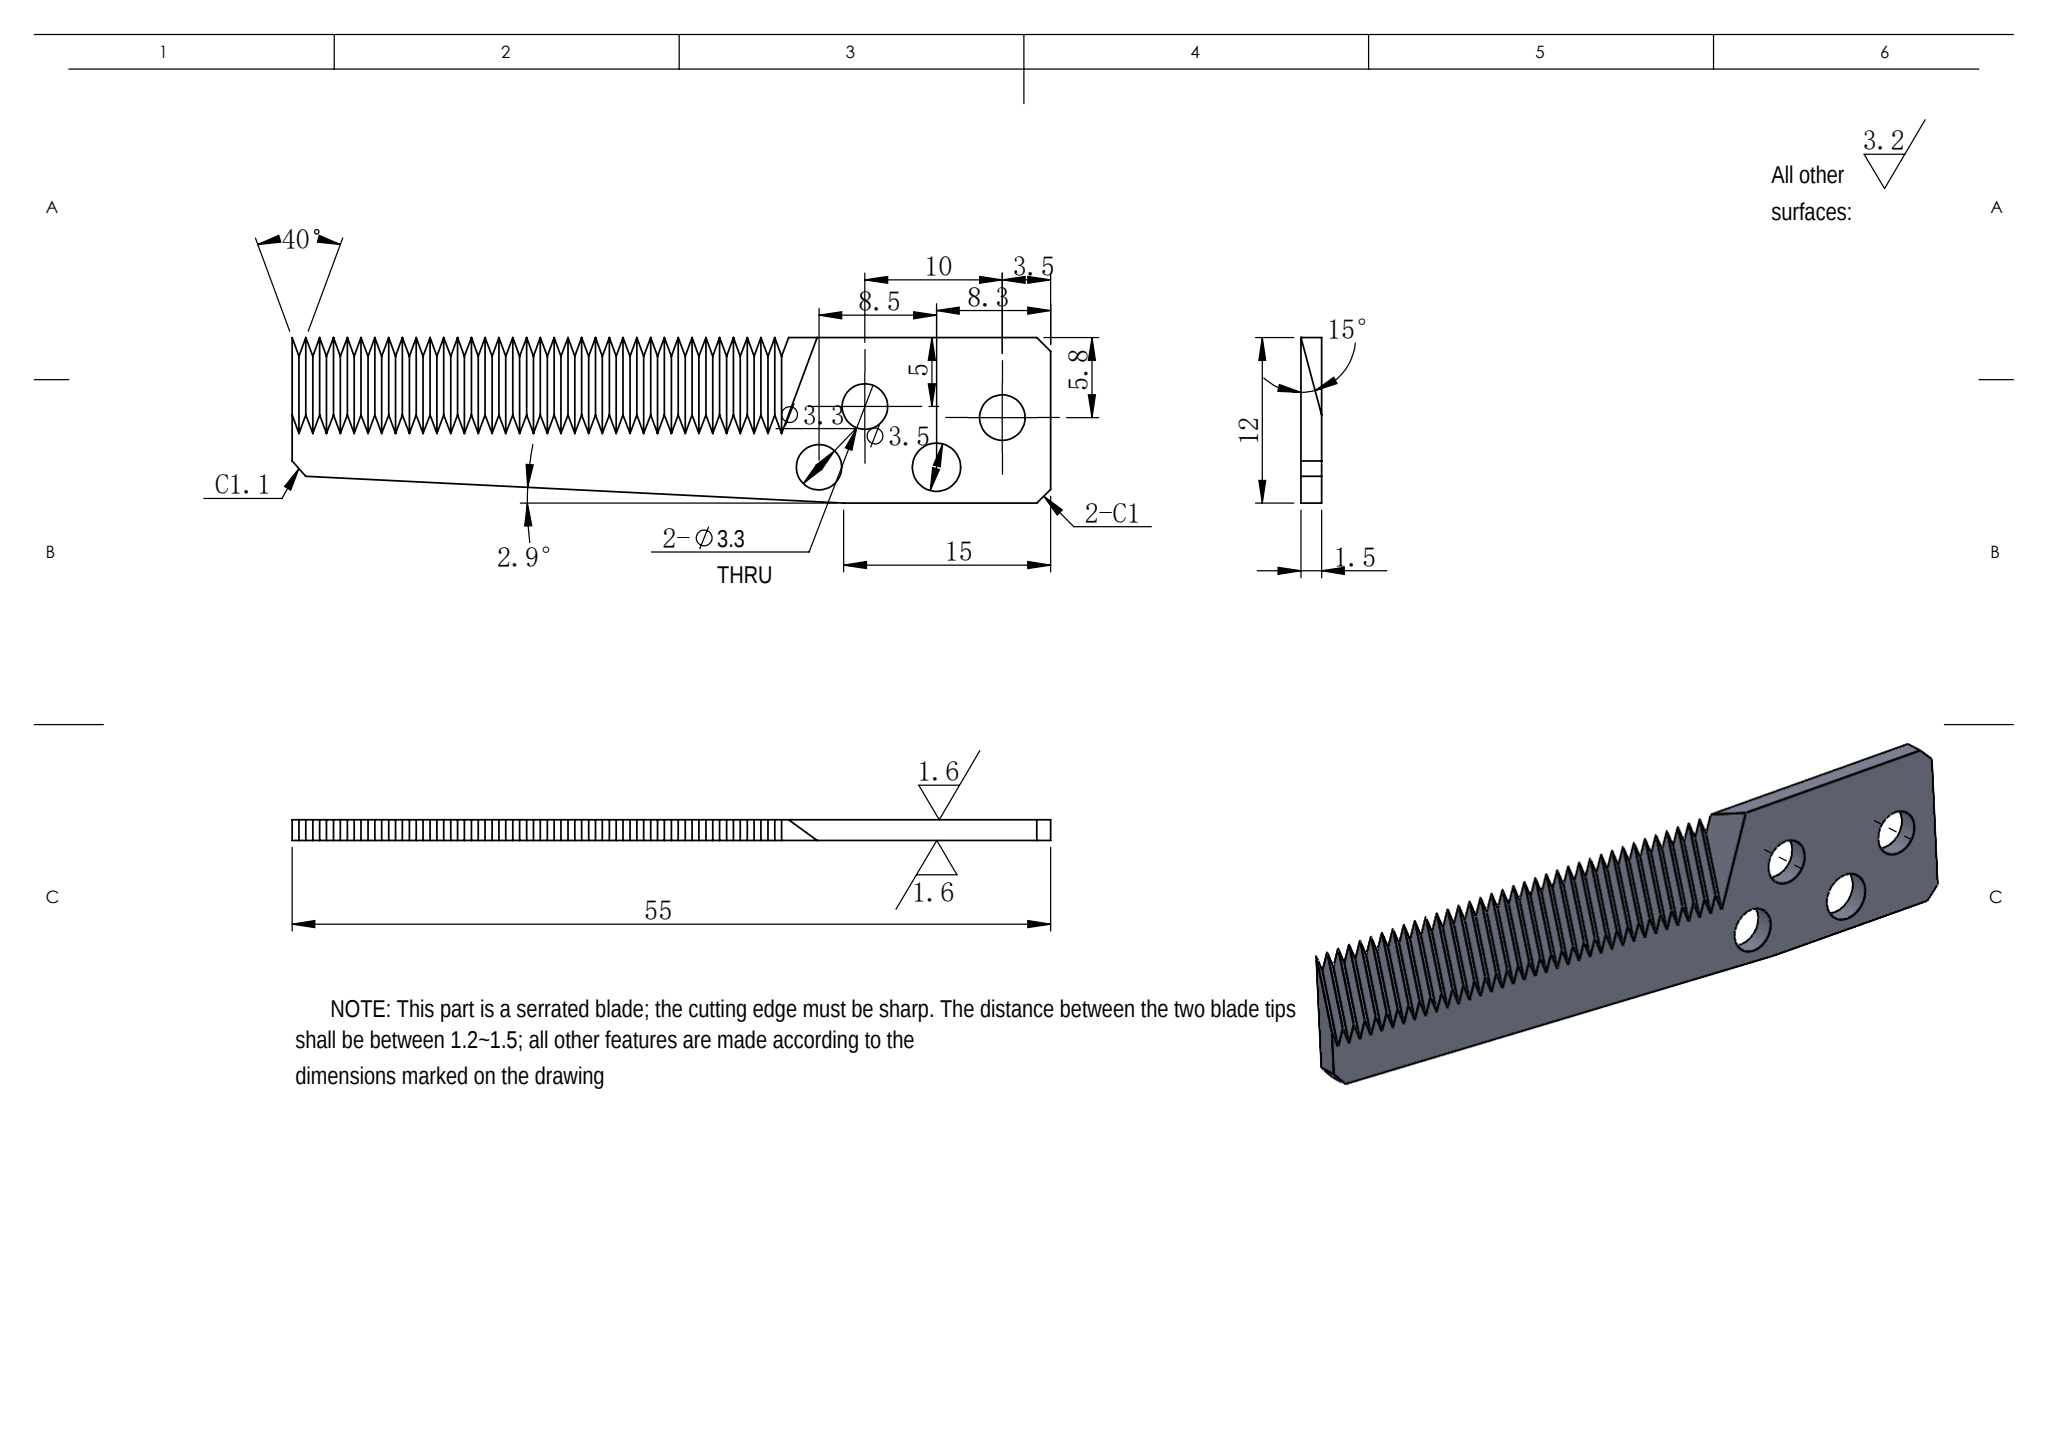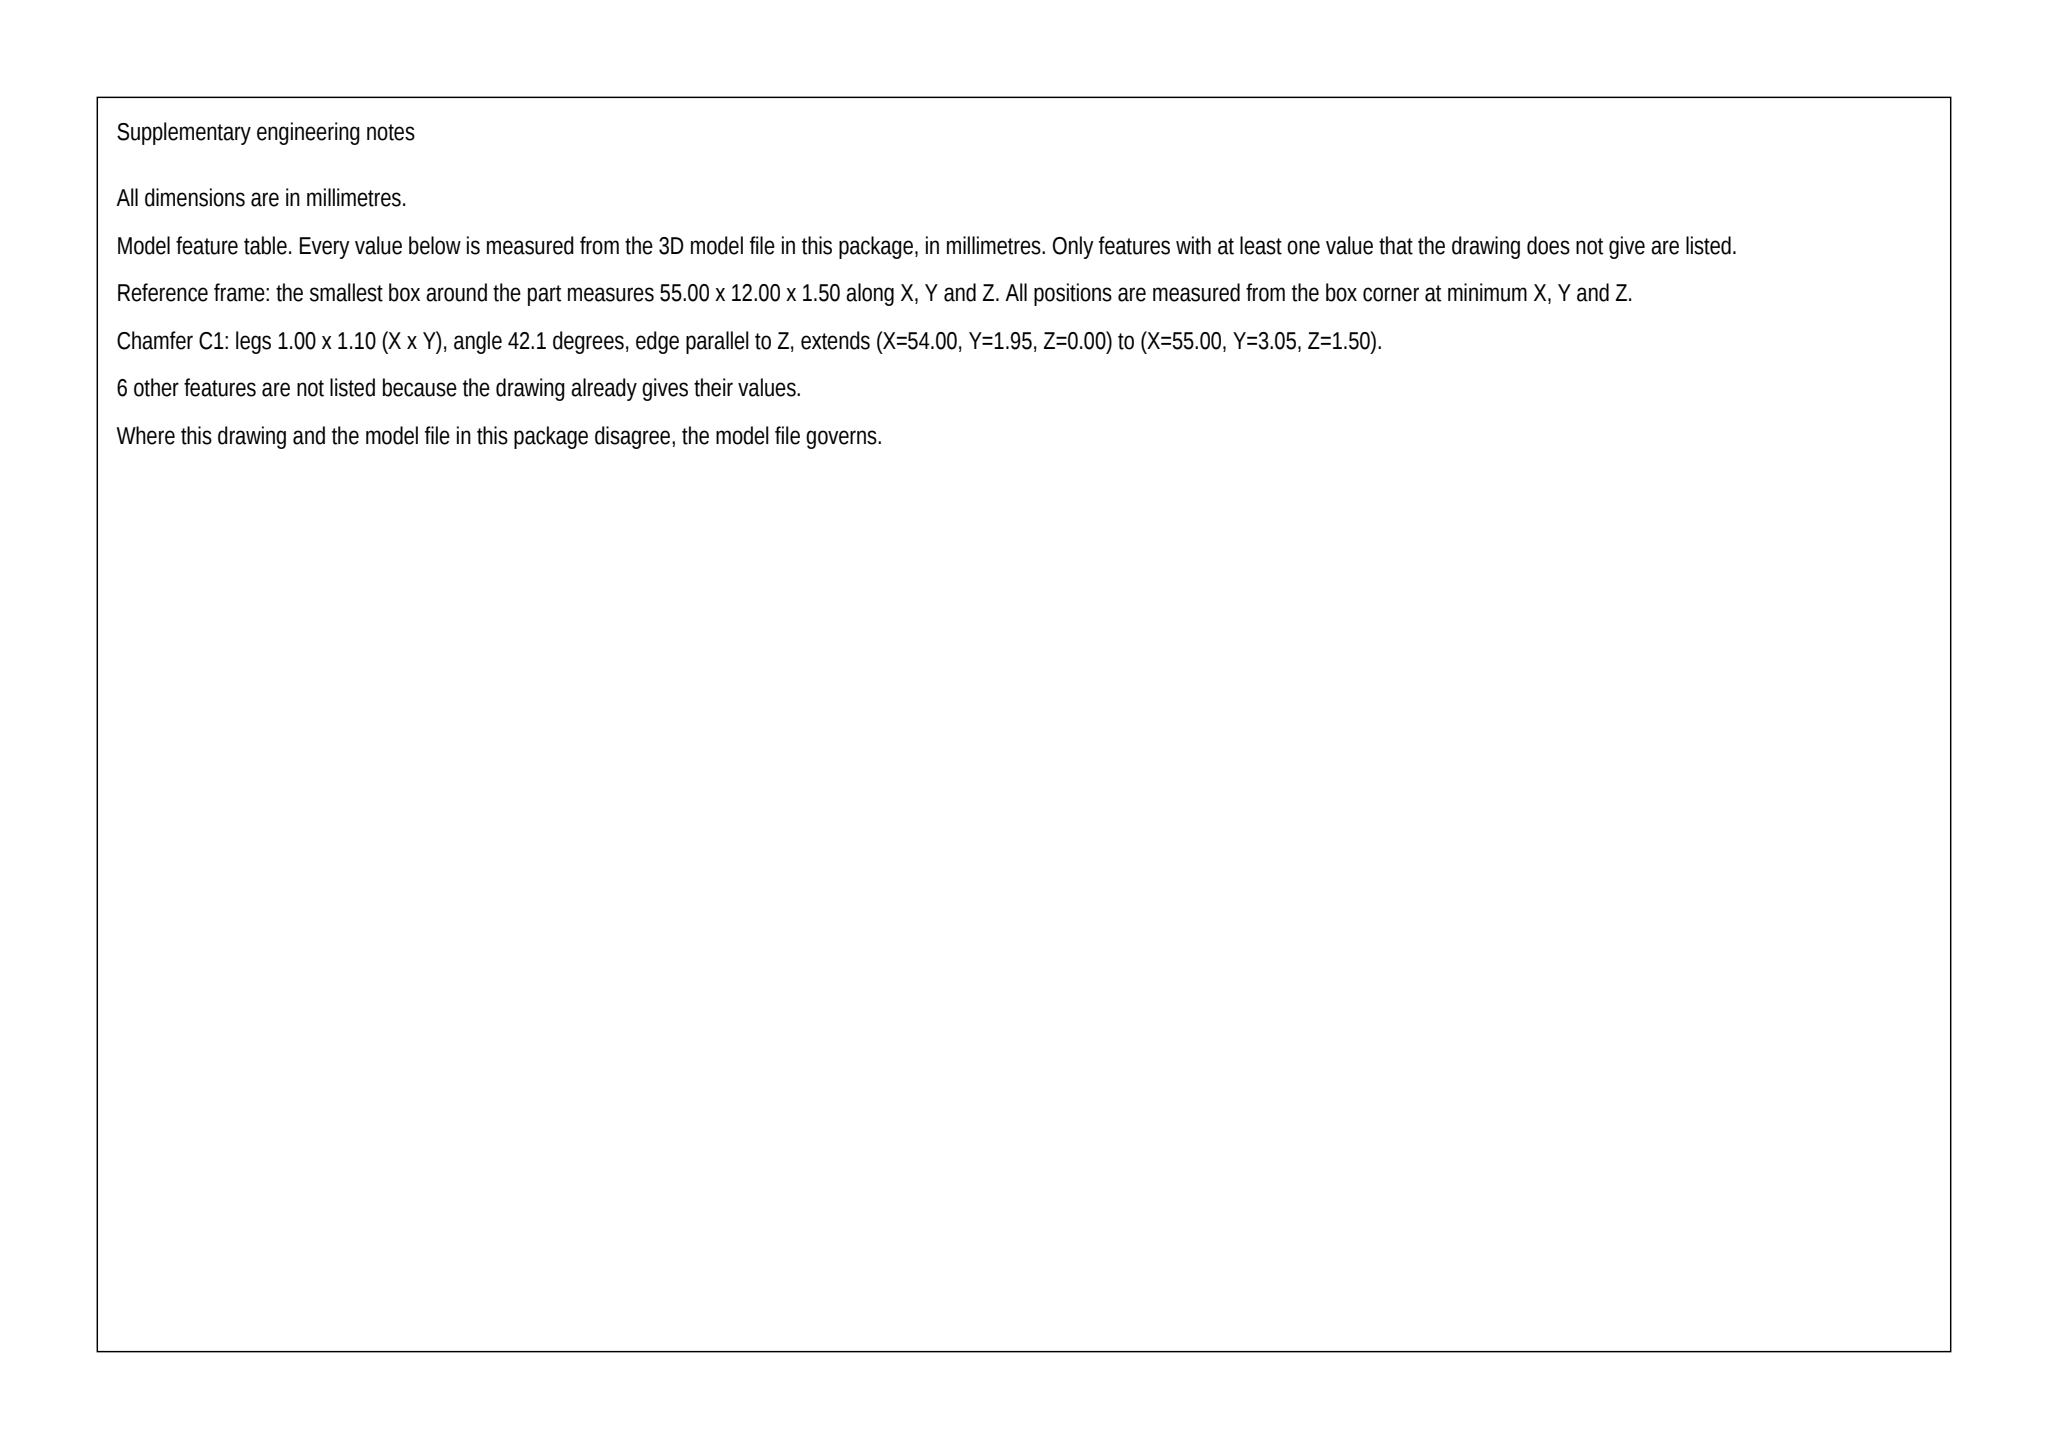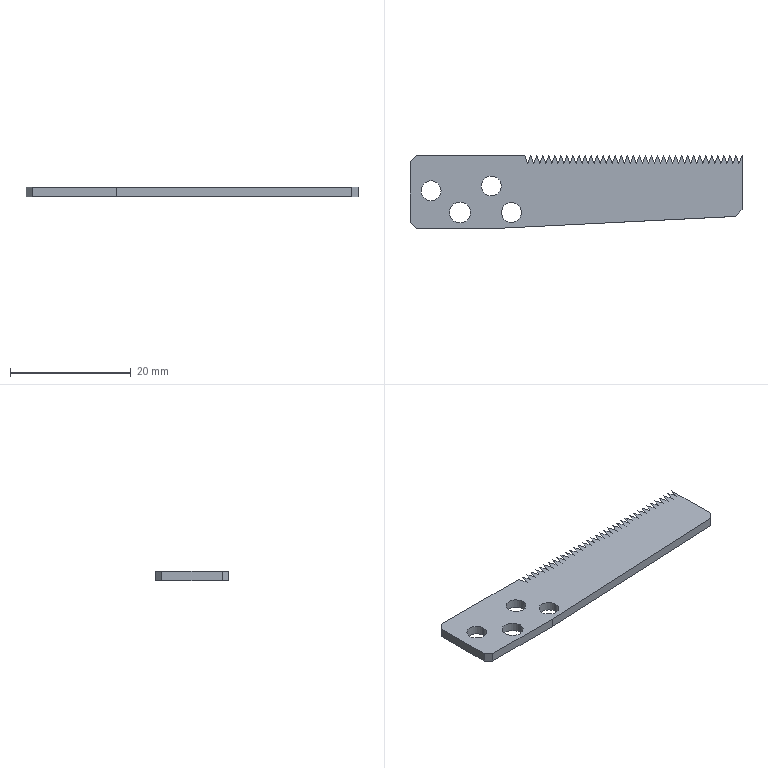Part | SolidWorks | mm | 1 solid | 90 faces | box 55 x 12 x 1.5 mm | volume 684 mm3 | plane 82 | cylinder 8 | commonest cylinder face diameters 3.3 x4 3.29 x2 3.501 x2
Drawing notes:
4 HOLE CL FM RH END: 3.5, 8.3, 13.5, 16.8 | from the solid: Z-axis cyl x = 3.5, 8.28, 13.47, 16.8 from bbox min corner (RH end face)
HOLE CL FM TOOTHED EDGE: 5.8, 9.4, 5.0, 9.4 RESP | from the solid: Cyl y = 6.2, 2.6, 7.0, 2.6; width 12 -> 5.8, 9.4, 5.0, 9.4 from y=12 edge
Ø3.5 THRU AT 8.3 FM RH END; OTHER 3 HOLES Ø3.3 THRU | from the solid: dia 3.501 at (8.28,2.6); dia 3.3/3.29 at (3.5,6.2),(13.47,7.0),(16.8,2.6), len 1.5 thru plate
SERRATED EDGE START: toothed section begins 19.5 from the holed end (X=19.5); transition run-out face spans X=16.9 to X=19.5 (2.6 long), flank/run-out faces inclined 55° to the length axis (77.8° to width, 37.7° to thickness). | from the solid: inclined_planes: [55.0,77.8,37.7] bbox_from [16.9,5.0,0.0] size [2.6,7.0,1.5]; first full flank bbox_from [19.5,5.0,0.0] size [0.5,7.0,1.5]
TOOTH FORM: serration flank faces run from root at Y=5.0 to tip at Y=12.0 on the toothed edge (7.0 root-to-tip height), full 1.5 thickness; flank faces repeat at 0.5 spacing along the length. | from the solid: inclined_planes [55.0,77.8,37.7] repeated at X=19.5,20.0,20.5...29.5, each size [0.5,7.0,1.5] with y extent 5.0-12.0; axis_planes y=12.0 (toothed edge) and bbox_xyz width 12.0
build123d program:
from build123d import *
from OCP.BRepFilletAPI import BRepFilletAPI_MakeChamfer

# Parameters (mm, degrees)
SKETCH2_W           = 55
SKETCH2_H           = 12
BOSS_EXTRUDE1_DEPTH = 1.5
CUT_EXTRUDE1_DEPTH  = 57.314
LPATTERN1_COUNT     = 36
LPATTERN1_PITCH     = 1
CUT_EXTRUDE2_DEPTH  = 57.314
SKETCH5_R           = 1.65
CUT_EXTRUDE3_DEPTH  = 57.314
CHAMFER1_SIZE       = 1
CHAMFER1_SIZE2      = 1.054
SKETCH6_R           = 1.645
SKETCH6_R_2         = 1.75
CUT_EXTRUDE4_DEPTH  = 10


with BuildPart() as part:
    # Sketch2 → Boss-Extrude1 (new body)
    with BuildSketch(Plane.XY):
        with Locations((27.5, 6)):
            Rectangle(SKETCH2_W, SKETCH2_H)
    extrude(amount=BOSS_EXTRUDE1_DEPTH)

    # Sketch3 → Cut-Extrude1 (cut, symmetric)
    with BuildSketch(Plane(origin=(0, 0, 0), x_dir=(-1, 0, 0), z_dir=(0, 0.9659, 0.2588))):
        Polygon((51.229, -75.338), (-51.5, -3.406), (-54.5, -1.306), (-57.5, -3.406), (-160.229, -75.338), (-160.229, -326.157), (51.229, -326.157), align=None)
    cut_extrude1 = extrude(amount=CUT_EXTRUDE1_DEPTH, both=True, mode=Mode.SUBTRACT)

    # LPattern1: Cut-Extrude1 ×36
    with Locations(*[(-i * LPATTERN1_PITCH, 0, 0) for i in range(1, LPATTERN1_COUNT)]):
        add(cut_extrude1, mode=Mode.SUBTRACT)

    # Sketch4 → Cut-Extrude2 (cut, through all)
    with BuildSketch(Plane(origin=(0, 0, 0), x_dir=(-1, 0, 0), z_dir=(0, 0, -1))):
        Polygon((-55, 2), (-15, 0), (-55, 0), align=None)
    extrude(amount=-CUT_EXTRUDE2_DEPTH, mode=Mode.SUBTRACT)

    # Sketch5 → Cut-Extrude3 (cut, through all)
    with BuildSketch(Plane(origin=(0, 0, 0), x_dir=(-1, 0, 0), z_dir=(0, 0, -1))):
        with Locations((-13.468, 7)):
            Circle(SKETCH5_R)
        with Locations((-3.5, 6.2)):
            Circle(SKETCH5_R)
    extrude(amount=-CUT_EXTRUDE3_DEPTH, mode=Mode.SUBTRACT)

    # Chamfer1: one chamfer whose edges measure the first distance from different faces: ONE call of the kernel's chamfer builder (chamfer() names one face for all edges)
    chamfer1_edges_1 = [part.edges().sort_by_distance(p)[0] for p in [
        (55, 2, 0.75),
    ]]
    chamfer1_side_1 = [part.faces().sort_by_distance(p)[0] for p in [
        (35, 1, 0.75),
    ]]
    chamfer1_edges_2 = [part.edges().sort_by_distance(p)[0] for p in [
        (0, 12, 0.75),
        (0, 0, 0.75),
    ]]
    chamfer1 = BRepFilletAPI_MakeChamfer(part.part.solid().wrapped)
    for e in chamfer1_edges_1:
        chamfer1.Add(CHAMFER1_SIZE, CHAMFER1_SIZE2, e.wrapped, chamfer1_side_1[0].wrapped)  # the first distance lies on this face
    for e in chamfer1_edges_2:
        chamfer1.Add(CHAMFER1_SIZE, e.wrapped)
    add(Compound.cast(chamfer1.Shape()), mode=Mode.REPLACE)

    # Sketch6 → Cut-Extrude4 (cut)
    with BuildSketch(Plane(origin=(0, 0, 0), x_dir=(-1, 0, 0), z_dir=(0, 0, -1))):
        with Locations((-16.797, 2.604)):
            Circle(SKETCH6_R)
        with Locations((-8.276, 2.604)):
            Circle(SKETCH6_R_2)
    extrude(amount=-CUT_EXTRUDE4_DEPTH, mode=Mode.SUBTRACT)


solid = part.part